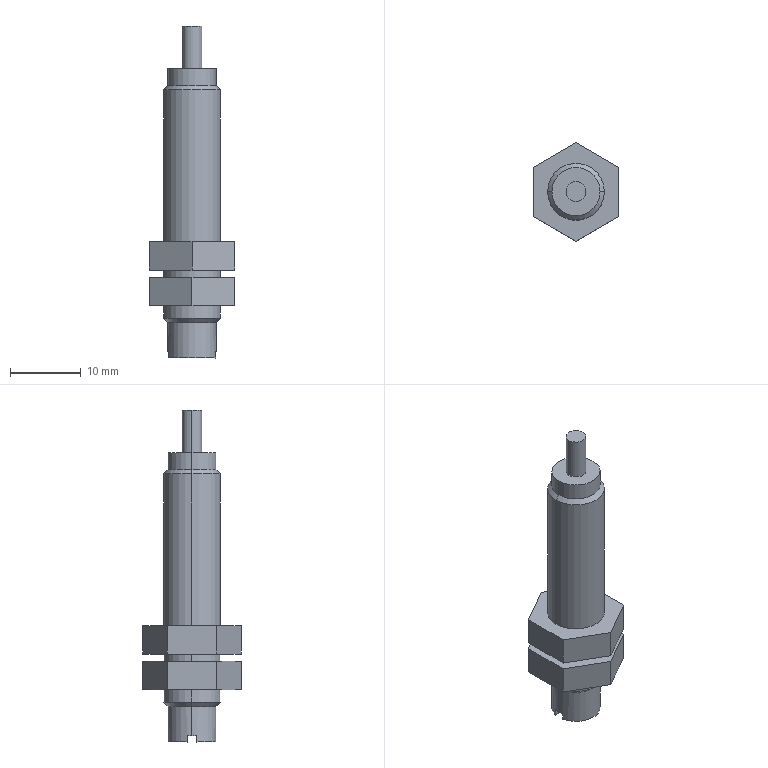Component | SolidWorks | RB0806-2 | 1 solid | 39 faces | box 12 x 13.86 x 46.8 mm | volume 2563 mm3 | plane 23 | cylinder 12 | cone 4 | commonest cylinder face diameters 8 x6 6.8 x4 2.8 x2
STEP:
#1=CARTESIAN_POINT('',(39.223,14.771,-15.48));
#2=VERTEX_POINT('',#1);
#3=CARTESIAN_POINT('',(39.538,14.771,-15.48));
#4=VERTEX_POINT('',#3);
#5=CARTESIAN_POINT('',(39.38,14.771,-15.48));
#6=DIRECTION('',(-0.00002551,-0.,-1.));
#7=DIRECTION('',(-1.,0.,0.00002551));
#8=AXIS2_PLACEMENT_3D('',#5,#6,#7);
#9=CIRCLE('',#8,0.1575);
#10=EDGE_CURVE('',#2,#4,#9,.T.);
#11=ORIENTED_EDGE('',*,*,#10,.F.);
#12=CARTESIAN_POINT('',(39.223,14.771,-14.638));
#13=VERTEX_POINT('',#12);
#14=CARTESIAN_POINT('',(39.223,14.771,-14.638));
#15=DIRECTION('',(0.00002551,0.,1.));
#16=VECTOR('',#15,39.37);
#17=LINE('',#14,#16);
#18=EDGE_CURVE('',#2,#13,#17,.T.);
#19=ORIENTED_EDGE('',*,*,#18,.T.);
#20=CARTESIAN_POINT('',(39.538,14.771,-14.638));
#21=VERTEX_POINT('',#20);
#22=CARTESIAN_POINT('',(39.38,14.771,-14.638));
#23=DIRECTION('',(0.00002551,0.,1.));
#24=DIRECTION('',(0.,1.,0.));
#25=AXIS2_PLACEMENT_3D('',#22,#23,#24);
#26=CIRCLE('',#25,0.1575);
#27=EDGE_CURVE('',#21,#13,#26,.T.);
#28=ORIENTED_EDGE('',*,*,#27,.F.);
#29=CARTESIAN_POINT('',(39.538,14.771,-14.638));
#30=DIRECTION('',(0.00002551,0.,1.));
#31=VECTOR('',#30,39.37);
#32=LINE('',#29,#31);
#33=EDGE_CURVE('',#4,#21,#32,.T.);
#34=ORIENTED_EDGE('',*,*,#33,.F.);
#35=EDGE_LOOP('',(#11,#19,#28,#34));
#36=FACE_OUTER_BOUND('',#35,.T.);
#37=CARTESIAN_POINT('',(39.38,14.771,-14.638));
#38=DIRECTION('',(0.00002551,0.,1.));
#39=DIRECTION('',(1.,0.,-0.00002551));
#40=AXIS2_PLACEMENT_3D('',#37,#38,#39);
#41=CYLINDRICAL_SURFACE('',#40,0.1575);
#42=ADVANCED_FACE('',(#36),#41,.T.);
#43=CARTESIAN_POINT('',(39.514,14.771,-14.614));
#44=VERTEX_POINT('',#43);
#45=CARTESIAN_POINT('',(39.247,14.771,-14.614));
#46=VERTEX_POINT('',#45);
#47=CARTESIAN_POINT('',(39.38,14.771,-14.614));
#48=DIRECTION('',(0.00002551,0.,1.));
#49=DIRECTION('',(0.,1.,0.));
#50=AXIS2_PLACEMENT_3D('',#47,#48,#49);
#51=CIRCLE('',#50,0.1339);
#52=EDGE_CURVE('',#44,#46,#51,.T.);
#53=ORIENTED_EDGE('',*,*,#52,.F.);
#54=CARTESIAN_POINT('',(39.514,14.771,-14.614));
#55=DIRECTION('',(0.7071,-0.,-0.7071));
#56=VECTOR('',#55,39.37);
#57=LINE('',#54,#56);
#58=EDGE_CURVE('',#44,#21,#57,.T.);
#59=ORIENTED_EDGE('',*,*,#58,.T.);
#60=ORIENTED_EDGE('',*,*,#27,.T.);
#61=CARTESIAN_POINT('',(39.247,14.771,-14.614));
#62=DIRECTION('',(-0.7071,-0.,-0.7071));
#63=VECTOR('',#62,39.37);
#64=LINE('',#61,#63);
#65=EDGE_CURVE('',#46,#13,#64,.T.);
#66=ORIENTED_EDGE('',*,*,#65,.F.);
#67=EDGE_LOOP('',(#53,#59,#60,#66));
#68=FACE_OUTER_BOUND('',#67,.T.);
#69=CARTESIAN_POINT('',(39.38,14.771,-14.614));
#70=DIRECTION('',(-0.00002551,-0.,-1.));
#71=DIRECTION('',(-1.,0.,0.00002551));
#72=AXIS2_PLACEMENT_3D('',#69,#70,#71);
#73=CONICAL_SURFACE('',#72,0.1339,0.7854);
#74=ADVANCED_FACE('',(#68),#73,.T.);
#75=ORIENTED_EDGE('',*,*,#52,.T.);
#76=CARTESIAN_POINT('',(39.247,14.771,-14.52));
#77=VERTEX_POINT('',#76);
#78=CARTESIAN_POINT('',(39.247,14.771,-14.52));
#79=DIRECTION('',(0.00002551,0.,1.));
#80=VECTOR('',#79,39.37);
#81=LINE('',#78,#80);
#82=EDGE_CURVE('',#46,#77,#81,.T.);
#83=ORIENTED_EDGE('',*,*,#82,.T.);
#84=CARTESIAN_POINT('',(39.514,14.771,-14.52));
#85=VERTEX_POINT('',#84);
#86=CARTESIAN_POINT('',(39.38,14.771,-14.52));
#87=DIRECTION('',(0.00002551,0.,1.));
#88=DIRECTION('',(1.,0.,-0.00002551));
#89=AXIS2_PLACEMENT_3D('',#86,#87,#88);
#90=CIRCLE('',#89,0.1339);
#91=EDGE_CURVE('',#85,#77,#90,.T.);
#92=ORIENTED_EDGE('',*,*,#91,.F.);
#93=CARTESIAN_POINT('',(39.514,14.771,-14.52));
#94=DIRECTION('',(0.00002551,0.,1.));
#95=VECTOR('',#94,39.37);
#96=LINE('',#93,#95);
#97=EDGE_CURVE('',#44,#85,#96,.T.);
#98=ORIENTED_EDGE('',*,*,#97,.F.);
#99=EDGE_LOOP('',(#75,#83,#92,#98));
#100=FACE_OUTER_BOUND('',#99,.T.);
#101=CARTESIAN_POINT('',(39.38,14.771,-14.52));
#102=DIRECTION('',(0.00002551,0.,1.));
#103=DIRECTION('',(1.,0.,-0.00002551));
#104=AXIS2_PLACEMENT_3D('',#101,#102,#103);
#105=CYLINDRICAL_SURFACE('',#104,0.1339);
#106=ADVANCED_FACE('',(#100),#105,.T.);
#107=CARTESIAN_POINT('',(39.436,14.771,-14.52));
#108=VERTEX_POINT('',#107);
#109=CARTESIAN_POINT('',(39.325,14.771,-14.52));
#110=VERTEX_POINT('',#109);
#111=CARTESIAN_POINT('',(39.38,14.771,-14.52));
#112=DIRECTION('',(0.00002551,0.,1.));
#113=DIRECTION('',(1.,0.,-0.00002551));
#114=AXIS2_PLACEMENT_3D('',#111,#112,#113);
#115=CIRCLE('',#114,0.05512);
#116=EDGE_CURVE('',#108,#110,#115,.T.);
#117=ORIENTED_EDGE('',*,*,#116,.T.);
#118=CARTESIAN_POINT('',(39.325,14.771,-14.283));
#119=VERTEX_POINT('',#118);
#120=CARTESIAN_POINT('',(39.325,14.771,-14.283));
#121=DIRECTION('',(0.00002551,0.,1.));
#122=VECTOR('',#121,39.37);
#123=LINE('',#120,#122);
#124=EDGE_CURVE('',#110,#119,#123,.T.);
#125=ORIENTED_EDGE('',*,*,#124,.T.);
#126=CARTESIAN_POINT('',(39.436,14.771,-14.283));
#127=VERTEX_POINT('',#126);
#128=CARTESIAN_POINT('',(39.38,14.771,-14.283));
#129=DIRECTION('',(-0.00002551,-0.,-1.));
#130=DIRECTION('',(1.,0.,-0.00002551));
#131=AXIS2_PLACEMENT_3D('',#128,#129,#130);
#132=CIRCLE('',#131,0.05512);
#133=EDGE_CURVE('',#119,#127,#132,.T.);
#134=ORIENTED_EDGE('',*,*,#133,.T.);
#135=CARTESIAN_POINT('',(39.436,14.771,-14.283));
#136=DIRECTION('',(0.00002551,0.,1.));
#137=VECTOR('',#136,39.37);
#138=LINE('',#135,#137);
#139=EDGE_CURVE('',#108,#127,#138,.T.);
#140=ORIENTED_EDGE('',*,*,#139,.F.);
#141=EDGE_LOOP('',(#117,#125,#134,#140));
#142=FACE_OUTER_BOUND('',#141,.T.);
#143=CARTESIAN_POINT('',(39.38,14.771,-14.283));
#144=DIRECTION('',(0.00002551,0.,1.));
#145=DIRECTION('',(1.,0.,-0.00002551));
#146=AXIS2_PLACEMENT_3D('',#143,#144,#145);
#147=CYLINDRICAL_SURFACE('',#146,0.05512);
#148=ADVANCED_FACE('',(#142),#147,.T.);
#149=CARTESIAN_POINT('',(39.538,14.771,-15.905));
#150=VERTEX_POINT('',#149);
#151=CARTESIAN_POINT('',(39.223,14.771,-15.905));
#152=VERTEX_POINT('',#151);
#153=CARTESIAN_POINT('',(39.38,14.771,-15.905));
#154=DIRECTION('',(0.00002551,0.,1.));
#155=DIRECTION('',(0.,1.,0.));
#156=AXIS2_PLACEMENT_3D('',#153,#154,#155);
#157=CIRCLE('',#156,0.1575);
#158=EDGE_CURVE('',#150,#152,#157,.T.);
#159=ORIENTED_EDGE('',*,*,#158,.T.);
#160=CARTESIAN_POINT('',(39.223,14.771,-15.835));
#161=VERTEX_POINT('',#160);
#162=CARTESIAN_POINT('',(39.223,14.771,-15.48));
#163=DIRECTION('',(0.00002551,0.,1.));
#164=VECTOR('',#163,39.37);
#165=LINE('',#162,#164);
#166=EDGE_CURVE('',#152,#161,#165,.T.);
#167=ORIENTED_EDGE('',*,*,#166,.T.);
#168=CARTESIAN_POINT('',(39.538,14.771,-15.835));
#169=VERTEX_POINT('',#168);
#170=CARTESIAN_POINT('',(39.38,14.771,-15.835));
#171=DIRECTION('',(-0.00002551,-0.,-1.));
#172=DIRECTION('',(1.,0.,-0.00002551));
#173=AXIS2_PLACEMENT_3D('',#170,#171,#172);
#174=CIRCLE('',#173,0.1575);
#175=EDGE_CURVE('',#161,#169,#174,.T.);
#176=ORIENTED_EDGE('',*,*,#175,.T.);
#177=CARTESIAN_POINT('',(39.538,14.771,-15.48));
#178=DIRECTION('',(0.00002551,0.,1.));
#179=VECTOR('',#178,39.37);
#180=LINE('',#177,#179);
#181=EDGE_CURVE('',#150,#169,#180,.T.);
#182=ORIENTED_EDGE('',*,*,#181,.F.);
#183=EDGE_LOOP('',(#159,#167,#176,#182));
#184=FACE_OUTER_BOUND('',#183,.T.);
#185=CARTESIAN_POINT('',(39.38,14.771,-15.48));
#186=DIRECTION('',(0.00002551,0.,1.));
#187=DIRECTION('',(1.,0.,-0.00002551));
#188=AXIS2_PLACEMENT_3D('',#185,#186,#187);
#189=CYLINDRICAL_SURFACE('',#188,0.1575);
#190=ADVANCED_FACE('',(#184),#189,.T.);
#191=CARTESIAN_POINT('',(39.514,14.771,-15.929));
#192=VERTEX_POINT('',#191);
#193=CARTESIAN_POINT('',(39.247,14.771,-15.929));
#194=VERTEX_POINT('',#193);
#195=CARTESIAN_POINT('',(39.38,14.771,-15.929));
#196=DIRECTION('',(0.00002551,0.,1.));
#197=DIRECTION('',(0.,1.,0.));
#198=AXIS2_PLACEMENT_3D('',#195,#196,#197);
#199=CIRCLE('',#198,0.1339);
#200=EDGE_CURVE('',#192,#194,#199,.T.);
#201=ORIENTED_EDGE('',*,*,#200,.T.);
#202=CARTESIAN_POINT('',(39.247,14.771,-15.929));
#203=DIRECTION('',(-0.7071,0.,0.7071));
#204=VECTOR('',#203,39.37);
#205=LINE('',#202,#204);
#206=EDGE_CURVE('',#194,#152,#205,.T.);
#207=ORIENTED_EDGE('',*,*,#206,.T.);
#208=ORIENTED_EDGE('',*,*,#158,.F.);
#209=CARTESIAN_POINT('',(39.514,14.771,-15.929));
#210=DIRECTION('',(0.7071,0.,0.7071));
#211=VECTOR('',#210,39.37);
#212=LINE('',#209,#211);
#213=EDGE_CURVE('',#192,#150,#212,.T.);
#214=ORIENTED_EDGE('',*,*,#213,.F.);
#215=EDGE_LOOP('',(#201,#207,#208,#214));
#216=FACE_OUTER_BOUND('',#215,.T.);
#217=CARTESIAN_POINT('',(39.38,14.771,-15.929));
#218=DIRECTION('',(0.00002551,0.,1.));
#219=DIRECTION('',(1.,0.,-0.00002551));
#220=AXIS2_PLACEMENT_3D('',#217,#218,#219);
#221=CONICAL_SURFACE('',#220,0.1339,0.7854);
#222=ADVANCED_FACE('',(#216),#221,.T.);
#223=CARTESIAN_POINT('',(39.247,14.771,-16.09));
#224=VERTEX_POINT('',#223);
#225=CARTESIAN_POINT('',(39.249,14.799,-16.09));
#226=VERTEX_POINT('',#225);
#227=CARTESIAN_POINT('',(39.38,14.771,-16.09));
#228=DIRECTION('',(-0.00002551,-0.,-1.));
#229=DIRECTION('',(1.,-0.,-0.00002551));
#230=AXIS2_PLACEMENT_3D('',#227,#228,#229);
#231=CIRCLE('',#230,0.1339);
#232=EDGE_CURVE('',#224,#226,#231,.T.);
#233=ORIENTED_EDGE('',*,*,#232,.F.);
#234=CARTESIAN_POINT('',(39.247,14.771,-15.929));
#235=DIRECTION('',(0.00002551,0.,1.));
#236=VECTOR('',#235,39.37);
#237=LINE('',#234,#236);
#238=EDGE_CURVE('',#224,#194,#237,.T.);
#239=ORIENTED_EDGE('',*,*,#238,.T.);
#240=ORIENTED_EDGE('',*,*,#200,.F.);
#241=CARTESIAN_POINT('',(39.514,14.771,-16.09));
#242=VERTEX_POINT('',#241);
#243=CARTESIAN_POINT('',(39.514,14.771,-15.929));
#244=DIRECTION('',(0.00002551,0.,1.));
#245=VECTOR('',#244,39.37);
#246=LINE('',#243,#245);
#247=EDGE_CURVE('',#242,#192,#246,.T.);
#248=ORIENTED_EDGE('',*,*,#247,.F.);
#249=CARTESIAN_POINT('',(39.511,14.799,-16.09));
#250=VERTEX_POINT('',#249);
#251=CARTESIAN_POINT('',(39.38,14.771,-16.09));
#252=DIRECTION('',(-0.00002551,-0.,-1.));
#253=DIRECTION('',(1.,-0.,-0.00002551));
#254=AXIS2_PLACEMENT_3D('',#251,#252,#253);
#255=CIRCLE('',#254,0.1339);
#256=EDGE_CURVE('',#250,#242,#255,.T.);
#257=ORIENTED_EDGE('',*,*,#256,.F.);
#258=CARTESIAN_POINT('',(39.511,14.799,-16.126));
#259=VERTEX_POINT('',#258);
#260=CARTESIAN_POINT('',(39.511,14.799,-16.108));
#261=DIRECTION('',(0.00002551,0.,1.));
#262=VECTOR('',#261,39.37);
#263=LINE('',#260,#262);
#264=EDGE_CURVE('',#259,#250,#263,.T.);
#265=ORIENTED_EDGE('',*,*,#264,.F.);
#266=CARTESIAN_POINT('',(39.249,14.799,-16.126));
#267=VERTEX_POINT('',#266);
#268=CARTESIAN_POINT('',(39.38,14.771,-16.126));
#269=DIRECTION('',(0.00002551,0.,1.));
#270=DIRECTION('',(1.,0.,-0.00002551));
#271=AXIS2_PLACEMENT_3D('',#268,#269,#270);
#272=CIRCLE('',#271,0.1339);
#273=EDGE_CURVE('',#259,#267,#272,.T.);
#274=ORIENTED_EDGE('',*,*,#273,.T.);
#275=CARTESIAN_POINT('',(39.249,14.799,-16.108));
#276=DIRECTION('',(-0.00002551,-0.,-1.));
#277=VECTOR('',#276,39.37);
#278=LINE('',#275,#277);
#279=EDGE_CURVE('',#226,#267,#278,.T.);
#280=ORIENTED_EDGE('',*,*,#279,.F.);
#281=EDGE_LOOP('',(#233,#239,#240,#248,#257,#265,#274,#280));
#282=FACE_OUTER_BOUND('',#281,.T.);
#283=CARTESIAN_POINT('',(39.38,14.771,-15.929));
#284=DIRECTION('',(0.00002551,0.,1.));
#285=DIRECTION('',(1.,0.,-0.00002551));
#286=AXIS2_PLACEMENT_3D('',#283,#284,#285);
#287=CYLINDRICAL_SURFACE('',#286,0.1339);
#288=ADVANCED_FACE('',(#282),#287,.T.);
#289=CARTESIAN_POINT('',(39.223,14.771,-15.677));
#290=VERTEX_POINT('',#289);
#291=CARTESIAN_POINT('',(39.538,14.771,-15.677));
#292=VERTEX_POINT('',#291);
#293=CARTESIAN_POINT('',(39.38,14.771,-15.677));
#294=DIRECTION('',(-0.00002551,-0.,-1.));
#295=DIRECTION('',(1.,-0.,-0.00002551));
#296=AXIS2_PLACEMENT_3D('',#293,#294,#295);
#297=CIRCLE('',#296,0.1575);
#298=EDGE_CURVE('',#290,#292,#297,.T.);
#299=ORIENTED_EDGE('',*,*,#298,.F.);
#300=CARTESIAN_POINT('',(39.223,14.771,-15.638));
#301=VERTEX_POINT('',#300);
#302=CARTESIAN_POINT('',(39.223,14.771,-15.48));
#303=DIRECTION('',(0.00002551,0.,1.));
#304=VECTOR('',#303,39.37);
#305=LINE('',#302,#304);
#306=EDGE_CURVE('',#290,#301,#305,.T.);
#307=ORIENTED_EDGE('',*,*,#306,.T.);
#308=CARTESIAN_POINT('',(39.538,14.771,-15.638));
#309=VERTEX_POINT('',#308);
#310=CARTESIAN_POINT('',(39.38,14.771,-15.638));
#311=DIRECTION('',(-0.00002551,-0.,-1.));
#312=DIRECTION('',(1.,-0.,-0.00002551));
#313=AXIS2_PLACEMENT_3D('',#310,#311,#312);
#314=CIRCLE('',#313,0.1575);
#315=EDGE_CURVE('',#301,#309,#314,.T.);
#316=ORIENTED_EDGE('',*,*,#315,.T.);
#317=CARTESIAN_POINT('',(39.538,14.771,-15.48));
#318=DIRECTION('',(0.00002551,0.,1.));
#319=VECTOR('',#318,39.37);
#320=LINE('',#317,#319);
#321=EDGE_CURVE('',#292,#309,#320,.T.);
#322=ORIENTED_EDGE('',*,*,#321,.F.);
#323=EDGE_LOOP('',(#299,#307,#316,#322));
#324=FACE_OUTER_BOUND('',#323,.T.);
#325=CARTESIAN_POINT('',(39.38,14.771,-15.48));
#326=DIRECTION('',(0.00002551,0.,1.));
#327=DIRECTION('',(1.,0.,-0.00002551));
#328=AXIS2_PLACEMENT_3D('',#325,#326,#327);
#329=CYLINDRICAL_SURFACE('',#328,0.1575);
#330=ADVANCED_FACE('',(#324),#329,.T.);
#331=CARTESIAN_POINT('',(39.38,15.044,-15.48));
#332=VERTEX_POINT('',#331);
#333=CARTESIAN_POINT('',(39.144,14.908,-15.48));
#334=VERTEX_POINT('',#333);
#335=CARTESIAN_POINT('',(39.144,14.908,-15.48));
#336=DIRECTION('',(-0.866,-0.5,0.00002209));
#337=VECTOR('',#336,39.37);
#338=LINE('',#335,#337);
#339=EDGE_CURVE('',#332,#334,#338,.T.);
#340=ORIENTED_EDGE('',*,*,#339,.F.);
#341=CARTESIAN_POINT('',(39.38,15.044,-15.638));
#342=VERTEX_POINT('',#341);
#343=CARTESIAN_POINT('',(39.38,15.044,-15.323));
#344=DIRECTION('',(-0.00002551,-0.,-1.));
#345=VECTOR('',#344,39.37);
#346=LINE('',#343,#345);
#347=EDGE_CURVE('',#332,#342,#346,.T.);
#348=ORIENTED_EDGE('',*,*,#347,.T.);
#349=CARTESIAN_POINT('',(39.144,14.908,-15.638));
#350=VERTEX_POINT('',#349);
#351=CARTESIAN_POINT('',(39.38,15.044,-15.638));
#352=DIRECTION('',(0.866,0.5,-0.00002209));
#353=VECTOR('',#352,39.37);
#354=LINE('',#351,#353);
#355=EDGE_CURVE('',#350,#342,#354,.T.);
#356=ORIENTED_EDGE('',*,*,#355,.F.);
#357=CARTESIAN_POINT('',(39.144,14.908,-15.323));
#358=DIRECTION('',(0.00002551,0.,1.));
#359=VECTOR('',#358,39.37);
#360=LINE('',#357,#359);
#361=EDGE_CURVE('',#350,#334,#360,.T.);
#362=ORIENTED_EDGE('',*,*,#361,.T.);
#363=EDGE_LOOP('',(#340,#348,#356,#362));
#364=FACE_OUTER_BOUND('',#363,.T.);
#365=CARTESIAN_POINT('',(39.144,14.908,-15.323));
#366=DIRECTION('',(-0.5,0.866,0.00001275));
#367=DIRECTION('',(0.866,0.5,-0.00002209));
#368=AXIS2_PLACEMENT_3D('',#365,#366,#367);
#369=PLANE('',#368);
#370=ADVANCED_FACE('',(#364),#369,.T.);
#371=CARTESIAN_POINT('',(39.617,14.908,-15.48));
#372=VERTEX_POINT('',#371);
#373=CARTESIAN_POINT('',(39.38,15.044,-15.48));
#374=DIRECTION('',(-0.866,0.5,0.00002209));
#375=VECTOR('',#374,39.37);
#376=LINE('',#373,#375);
#377=EDGE_CURVE('',#372,#332,#376,.T.);
#378=ORIENTED_EDGE('',*,*,#377,.F.);
#379=CARTESIAN_POINT('',(39.617,14.908,-15.638));
#380=VERTEX_POINT('',#379);
#381=CARTESIAN_POINT('',(39.617,14.908,-15.323));
#382=DIRECTION('',(-0.00002551,-0.,-1.));
#383=VECTOR('',#382,39.37);
#384=LINE('',#381,#383);
#385=EDGE_CURVE('',#372,#380,#384,.T.);
#386=ORIENTED_EDGE('',*,*,#385,.T.);
#387=CARTESIAN_POINT('',(39.617,14.908,-15.638));
#388=DIRECTION('',(0.866,-0.5,-0.00002209));
#389=VECTOR('',#388,39.37);
#390=LINE('',#387,#389);
#391=EDGE_CURVE('',#342,#380,#390,.T.);
#392=ORIENTED_EDGE('',*,*,#391,.F.);
#393=ORIENTED_EDGE('',*,*,#347,.F.);
#394=EDGE_LOOP('',(#378,#386,#392,#393));
#395=FACE_OUTER_BOUND('',#394,.T.);
#396=CARTESIAN_POINT('',(39.38,15.044,-15.323));
#397=DIRECTION('',(0.5,0.866,-0.00001275));
#398=DIRECTION('',(0.866,-0.5,-0.00002209));
#399=AXIS2_PLACEMENT_3D('',#396,#397,#398);
#400=PLANE('',#399);
#401=ADVANCED_FACE('',(#395),#400,.T.);
#402=CARTESIAN_POINT('',(39.617,14.635,-15.48));
#403=VERTEX_POINT('',#402);
#404=CARTESIAN_POINT('',(39.617,14.908,-15.48));
#405=DIRECTION('',(0.,1.,-0.));
#406=VECTOR('',#405,39.37);
#407=LINE('',#404,#406);
#408=EDGE_CURVE('',#403,#372,#407,.T.);
#409=ORIENTED_EDGE('',*,*,#408,.F.);
#410=CARTESIAN_POINT('',(39.617,14.635,-15.638));
#411=VERTEX_POINT('',#410);
#412=CARTESIAN_POINT('',(39.617,14.635,-15.323));
#413=DIRECTION('',(-0.00002551,-0.,-1.));
#414=VECTOR('',#413,39.37);
#415=LINE('',#412,#414);
#416=EDGE_CURVE('',#403,#411,#415,.T.);
#417=ORIENTED_EDGE('',*,*,#416,.T.);
#418=CARTESIAN_POINT('',(39.617,14.635,-15.638));
#419=DIRECTION('',(-0.,-1.,0.));
#420=VECTOR('',#419,39.37);
#421=LINE('',#418,#420);
#422=EDGE_CURVE('',#380,#411,#421,.T.);
#423=ORIENTED_EDGE('',*,*,#422,.F.);
#424=ORIENTED_EDGE('',*,*,#385,.F.);
#425=EDGE_LOOP('',(#409,#417,#423,#424));
#426=FACE_OUTER_BOUND('',#425,.T.);
#427=CARTESIAN_POINT('',(39.617,14.908,-15.323));
#428=DIRECTION('',(1.,-0.,-0.00002551));
#429=DIRECTION('',(-0.,-1.,0.));
#430=AXIS2_PLACEMENT_3D('',#427,#428,#429);
#431=PLANE('',#430);
#432=ADVANCED_FACE('',(#426),#431,.T.);
#433=CARTESIAN_POINT('',(39.38,14.499,-15.48));
#434=VERTEX_POINT('',#433);
#435=CARTESIAN_POINT('',(39.617,14.635,-15.48));
#436=DIRECTION('',(0.866,0.5,-0.00002209));
#437=VECTOR('',#436,39.37);
#438=LINE('',#435,#437);
#439=EDGE_CURVE('',#434,#403,#438,.T.);
#440=ORIENTED_EDGE('',*,*,#439,.F.);
#441=CARTESIAN_POINT('',(39.38,14.499,-15.638));
#442=VERTEX_POINT('',#441);
#443=CARTESIAN_POINT('',(39.38,14.499,-15.323));
#444=DIRECTION('',(-0.00002551,-0.,-1.));
#445=VECTOR('',#444,39.37);
#446=LINE('',#443,#445);
#447=EDGE_CURVE('',#434,#442,#446,.T.);
#448=ORIENTED_EDGE('',*,*,#447,.T.);
#449=CARTESIAN_POINT('',(39.38,14.499,-15.638));
#450=DIRECTION('',(-0.866,-0.5,0.00002209));
#451=VECTOR('',#450,39.37);
#452=LINE('',#449,#451);
#453=EDGE_CURVE('',#411,#442,#452,.T.);
#454=ORIENTED_EDGE('',*,*,#453,.F.);
#455=ORIENTED_EDGE('',*,*,#416,.F.);
#456=EDGE_LOOP('',(#440,#448,#454,#455));
#457=FACE_OUTER_BOUND('',#456,.T.);
#458=CARTESIAN_POINT('',(39.617,14.635,-15.323));
#459=DIRECTION('',(0.5,-0.866,-0.00001275));
#460=DIRECTION('',(-0.866,-0.5,0.00002209));
#461=AXIS2_PLACEMENT_3D('',#458,#459,#460);
#462=PLANE('',#461);
#463=ADVANCED_FACE('',(#457),#462,.T.);
#464=CARTESIAN_POINT('',(39.144,14.635,-15.48));
#465=VERTEX_POINT('',#464);
#466=CARTESIAN_POINT('',(39.38,14.499,-15.48));
#467=DIRECTION('',(0.866,-0.5,-0.00002209));
#468=VECTOR('',#467,39.37);
#469=LINE('',#466,#468);
#470=EDGE_CURVE('',#465,#434,#469,.T.);
#471=ORIENTED_EDGE('',*,*,#470,.F.);
#472=CARTESIAN_POINT('',(39.144,14.635,-15.638));
#473=VERTEX_POINT('',#472);
#474=CARTESIAN_POINT('',(39.144,14.635,-15.323));
#475=DIRECTION('',(-0.00002551,-0.,-1.));
#476=VECTOR('',#475,39.37);
#477=LINE('',#474,#476);
#478=EDGE_CURVE('',#465,#473,#477,.T.);
#479=ORIENTED_EDGE('',*,*,#478,.T.);
#480=CARTESIAN_POINT('',(39.144,14.635,-15.638));
#481=DIRECTION('',(-0.866,0.5,0.00002209));
#482=VECTOR('',#481,39.37);
#483=LINE('',#480,#482);
#484=EDGE_CURVE('',#442,#473,#483,.T.);
#485=ORIENTED_EDGE('',*,*,#484,.F.);
#486=ORIENTED_EDGE('',*,*,#447,.F.);
#487=EDGE_LOOP('',(#471,#479,#485,#486));
#488=FACE_OUTER_BOUND('',#487,.T.);
#489=CARTESIAN_POINT('',(39.38,14.499,-15.323));
#490=DIRECTION('',(-0.5,-0.866,0.00001275));
#491=DIRECTION('',(-0.866,0.5,0.00002209));
#492=AXIS2_PLACEMENT_3D('',#489,#490,#491);
#493=PLANE('',#492);
#494=ADVANCED_FACE('',(#488),#493,.T.);
#495=CARTESIAN_POINT('',(39.144,14.635,-15.48));
#496=DIRECTION('',(-0.,-1.,0.));
#497=VECTOR('',#496,39.37);
#498=LINE('',#495,#497);
#499=EDGE_CURVE('',#334,#465,#498,.T.);
#500=ORIENTED_EDGE('',*,*,#499,.F.);
#501=ORIENTED_EDGE('',*,*,#361,.F.);
#502=CARTESIAN_POINT('',(39.144,14.908,-15.638));
#503=DIRECTION('',(0.,1.,-0.));
#504=VECTOR('',#503,39.37);
#505=LINE('',#502,#504);
#506=EDGE_CURVE('',#473,#350,#505,.T.);
#507=ORIENTED_EDGE('',*,*,#506,.F.);
#508=ORIENTED_EDGE('',*,*,#478,.F.);
#509=EDGE_LOOP('',(#500,#501,#507,#508));
#510=FACE_OUTER_BOUND('',#509,.T.);
#511=CARTESIAN_POINT('',(39.144,14.635,-15.323));
#512=DIRECTION('',(-1.,0.,0.00002551));
#513=DIRECTION('',(0.,1.,-0.));
#514=AXIS2_PLACEMENT_3D('',#511,#512,#513);
#515=PLANE('',#514);
#516=ADVANCED_FACE('',(#510),#515,.T.);
#517=CARTESIAN_POINT('',(39.38,14.771,-15.638));
#518=DIRECTION('',(-0.00002551,-0.,-1.));
#519=DIRECTION('',(1.,0.,-0.00002551));
#520=AXIS2_PLACEMENT_3D('',#517,#518,#519);
#521=CIRCLE('',#520,0.1575);
#522=EDGE_CURVE('',#309,#301,#521,.T.);
#523=ORIENTED_EDGE('',*,*,#522,.F.);
#524=ORIENTED_EDGE('',*,*,#315,.F.);
#525=EDGE_LOOP('',(#523,#524));
#526=FACE_BOUND('',#525,.T.);
#527=ORIENTED_EDGE('',*,*,#422,.T.);
#528=ORIENTED_EDGE('',*,*,#453,.T.);
#529=ORIENTED_EDGE('',*,*,#484,.T.);
#530=ORIENTED_EDGE('',*,*,#506,.T.);
#531=ORIENTED_EDGE('',*,*,#355,.T.);
#532=ORIENTED_EDGE('',*,*,#391,.T.);
#533=EDGE_LOOP('',(#527,#528,#529,#530,#531,#532));
#534=FACE_OUTER_BOUND('',#533,.T.);
#535=CARTESIAN_POINT('',(39.38,14.771,-15.638));
#536=DIRECTION('',(0.00002551,0.,1.));
#537=DIRECTION('',(1.,-0.,-0.00002551));
#538=AXIS2_PLACEMENT_3D('',#535,#536,#537);
#539=PLANE('',#538);
#540=ADVANCED_FACE('',(#526,#534),#539,.F.);
#541=ORIENTED_EDGE('',*,*,#306,.F.);
#542=CARTESIAN_POINT('',(39.38,14.771,-15.677));
#543=DIRECTION('',(-0.00002551,-0.,-1.));
#544=DIRECTION('',(1.,0.,-0.00002551));
#545=AXIS2_PLACEMENT_3D('',#542,#543,#544);
#546=CIRCLE('',#545,0.1575);
#547=EDGE_CURVE('',#292,#290,#546,.T.);
#548=ORIENTED_EDGE('',*,*,#547,.F.);
#549=ORIENTED_EDGE('',*,*,#321,.T.);
#550=ORIENTED_EDGE('',*,*,#522,.T.);
#551=EDGE_LOOP('',(#541,#548,#549,#550));
#552=FACE_OUTER_BOUND('',#551,.T.);
#553=CARTESIAN_POINT('',(39.38,14.771,-15.48));
#554=DIRECTION('',(0.00002551,0.,1.));
#555=DIRECTION('',(1.,0.,-0.00002551));
#556=AXIS2_PLACEMENT_3D('',#553,#554,#555);
#557=CYLINDRICAL_SURFACE('',#556,0.1575);
#558=ADVANCED_FACE('',(#552),#557,.T.);
#559=CARTESIAN_POINT('',(39.617,14.908,-15.677));
#560=VERTEX_POINT('',#559);
#561=CARTESIAN_POINT('',(39.617,14.635,-15.677));
#562=VERTEX_POINT('',#561);
#563=CARTESIAN_POINT('',(39.617,14.635,-15.677));
#564=DIRECTION('',(-0.,-1.,0.));
#565=VECTOR('',#564,39.37);
#566=LINE('',#563,#565);
#567=EDGE_CURVE('',#560,#562,#566,.T.);
#568=ORIENTED_EDGE('',*,*,#567,.T.);
#569=CARTESIAN_POINT('',(39.617,14.635,-15.835));
#570=VERTEX_POINT('',#569);
#571=CARTESIAN_POINT('',(39.617,14.635,-15.835));
#572=DIRECTION('',(0.00002551,0.,1.));
#573=VECTOR('',#572,39.37);
#574=LINE('',#571,#573);
#575=EDGE_CURVE('',#570,#562,#574,.T.);
#576=ORIENTED_EDGE('',*,*,#575,.F.);
#577=CARTESIAN_POINT('',(39.617,14.908,-15.835));
#578=VERTEX_POINT('',#577);
#579=CARTESIAN_POINT('',(39.617,14.635,-15.835));
#580=DIRECTION('',(-0.,-1.,0.));
#581=VECTOR('',#580,39.37);
#582=LINE('',#579,#581);
#583=EDGE_CURVE('',#578,#570,#582,.T.);
#584=ORIENTED_EDGE('',*,*,#583,.F.);
#585=CARTESIAN_POINT('',(39.617,14.908,-15.835));
#586=DIRECTION('',(0.00002551,0.,1.));
#587=VECTOR('',#586,39.37);
#588=LINE('',#585,#587);
#589=EDGE_CURVE('',#578,#560,#588,.T.);
#590=ORIENTED_EDGE('',*,*,#589,.T.);
#591=EDGE_LOOP('',(#568,#576,#584,#590));
#592=FACE_OUTER_BOUND('',#591,.T.);
#593=CARTESIAN_POINT('',(39.617,14.635,-15.835));
#594=DIRECTION('',(-1.,0.,0.00002551));
#595=DIRECTION('',(-0.,-1.,0.));
#596=AXIS2_PLACEMENT_3D('',#593,#594,#595);
#597=PLANE('',#596);
#598=ADVANCED_FACE('',(#592),#597,.F.);
#599=CARTESIAN_POINT('',(39.38,14.499,-15.677));
#600=VERTEX_POINT('',#599);
#601=CARTESIAN_POINT('',(39.38,14.499,-15.677));
#602=DIRECTION('',(-0.866,-0.5,0.00002209));
#603=VECTOR('',#602,39.37);
#604=LINE('',#601,#603);
#605=EDGE_CURVE('',#562,#600,#604,.T.);
#606=ORIENTED_EDGE('',*,*,#605,.T.);
#607=CARTESIAN_POINT('',(39.38,14.499,-15.835));
#608=VERTEX_POINT('',#607);
#609=CARTESIAN_POINT('',(39.38,14.499,-15.835));
#610=DIRECTION('',(0.00002551,0.,1.));
#611=VECTOR('',#610,39.37);
#612=LINE('',#609,#611);
#613=EDGE_CURVE('',#608,#600,#612,.T.);
#614=ORIENTED_EDGE('',*,*,#613,.F.);
#615=CARTESIAN_POINT('',(39.38,14.499,-15.835));
#616=DIRECTION('',(-0.866,-0.5,0.00002209));
#617=VECTOR('',#616,39.37);
#618=LINE('',#615,#617);
#619=EDGE_CURVE('',#570,#608,#618,.T.);
#620=ORIENTED_EDGE('',*,*,#619,.F.);
#621=ORIENTED_EDGE('',*,*,#575,.T.);
#622=EDGE_LOOP('',(#606,#614,#620,#621));
#623=FACE_OUTER_BOUND('',#622,.T.);
#624=CARTESIAN_POINT('',(39.38,14.499,-15.835));
#625=DIRECTION('',(-0.5,0.866,0.00001275));
#626=DIRECTION('',(-0.866,-0.5,0.00002209));
#627=AXIS2_PLACEMENT_3D('',#624,#625,#626);
#628=PLANE('',#627);
#629=ADVANCED_FACE('',(#623),#628,.F.);
#630=CARTESIAN_POINT('',(39.144,14.635,-15.677));
#631=VERTEX_POINT('',#630);
#632=CARTESIAN_POINT('',(39.144,14.635,-15.677));
#633=DIRECTION('',(-0.866,0.5,0.00002209));
#634=VECTOR('',#633,39.37);
#635=LINE('',#632,#634);
#636=EDGE_CURVE('',#600,#631,#635,.T.);
#637=ORIENTED_EDGE('',*,*,#636,.T.);
#638=CARTESIAN_POINT('',(39.144,14.635,-15.835));
#639=VERTEX_POINT('',#638);
#640=CARTESIAN_POINT('',(39.144,14.635,-15.835));
#641=DIRECTION('',(0.00002551,0.,1.));
#642=VECTOR('',#641,39.37);
#643=LINE('',#640,#642);
#644=EDGE_CURVE('',#639,#631,#643,.T.);
#645=ORIENTED_EDGE('',*,*,#644,.F.);
#646=CARTESIAN_POINT('',(39.144,14.635,-15.835));
#647=DIRECTION('',(-0.866,0.5,0.00002209));
#648=VECTOR('',#647,39.37);
#649=LINE('',#646,#648);
#650=EDGE_CURVE('',#608,#639,#649,.T.);
#651=ORIENTED_EDGE('',*,*,#650,.F.);
#652=ORIENTED_EDGE('',*,*,#613,.T.);
#653=EDGE_LOOP('',(#637,#645,#651,#652));
#654=FACE_OUTER_BOUND('',#653,.T.);
#655=CARTESIAN_POINT('',(39.144,14.635,-15.835));
#656=DIRECTION('',(0.5,0.866,-0.00001275));
#657=DIRECTION('',(-0.866,0.5,0.00002209));
#658=AXIS2_PLACEMENT_3D('',#655,#656,#657);
#659=PLANE('',#658);
#660=ADVANCED_FACE('',(#654),#659,.F.);
#661=CARTESIAN_POINT('',(39.144,14.908,-15.677));
#662=VERTEX_POINT('',#661);
#663=CARTESIAN_POINT('',(39.144,14.908,-15.677));
#664=DIRECTION('',(0.,1.,-0.));
#665=VECTOR('',#664,39.37);
#666=LINE('',#663,#665);
#667=EDGE_CURVE('',#631,#662,#666,.T.);
#668=ORIENTED_EDGE('',*,*,#667,.T.);
#669=CARTESIAN_POINT('',(39.144,14.908,-15.835));
#670=VERTEX_POINT('',#669);
#671=CARTESIAN_POINT('',(39.144,14.908,-15.835));
#672=DIRECTION('',(0.00002551,0.,1.));
#673=VECTOR('',#672,39.37);
#674=LINE('',#671,#673);
#675=EDGE_CURVE('',#670,#662,#674,.T.);
#676=ORIENTED_EDGE('',*,*,#675,.F.);
#677=CARTESIAN_POINT('',(39.144,14.908,-15.835));
#678=DIRECTION('',(0.,1.,-0.));
#679=VECTOR('',#678,39.37);
#680=LINE('',#677,#679);
#681=EDGE_CURVE('',#639,#670,#680,.T.);
#682=ORIENTED_EDGE('',*,*,#681,.F.);
#683=ORIENTED_EDGE('',*,*,#644,.T.);
#684=EDGE_LOOP('',(#668,#676,#682,#683));
#685=FACE_OUTER_BOUND('',#684,.T.);
#686=CARTESIAN_POINT('',(39.144,14.908,-15.835));
#687=DIRECTION('',(1.,-0.,-0.00002551));
#688=DIRECTION('',(0.,1.,-0.));
#689=AXIS2_PLACEMENT_3D('',#686,#687,#688);
#690=PLANE('',#689);
#691=ADVANCED_FACE('',(#685),#690,.F.);
#692=CARTESIAN_POINT('',(39.38,15.044,-15.677));
#693=VERTEX_POINT('',#692);
#694=CARTESIAN_POINT('',(39.38,15.044,-15.677));
#695=DIRECTION('',(0.866,0.5,-0.00002209));
#696=VECTOR('',#695,39.37);
#697=LINE('',#694,#696);
#698=EDGE_CURVE('',#662,#693,#697,.T.);
#699=ORIENTED_EDGE('',*,*,#698,.T.);
#700=CARTESIAN_POINT('',(39.38,15.044,-15.835));
#701=VERTEX_POINT('',#700);
#702=CARTESIAN_POINT('',(39.38,15.044,-15.835));
#703=DIRECTION('',(0.00002551,0.,1.));
#704=VECTOR('',#703,39.37);
#705=LINE('',#702,#704);
#706=EDGE_CURVE('',#701,#693,#705,.T.);
#707=ORIENTED_EDGE('',*,*,#706,.F.);
#708=CARTESIAN_POINT('',(39.38,15.044,-15.835));
#709=DIRECTION('',(0.866,0.5,-0.00002209));
#710=VECTOR('',#709,39.37);
#711=LINE('',#708,#710);
#712=EDGE_CURVE('',#670,#701,#711,.T.);
#713=ORIENTED_EDGE('',*,*,#712,.F.);
#714=ORIENTED_EDGE('',*,*,#675,.T.);
#715=EDGE_LOOP('',(#699,#707,#713,#714));
#716=FACE_OUTER_BOUND('',#715,.T.);
#717=CARTESIAN_POINT('',(39.38,15.044,-15.835));
#718=DIRECTION('',(0.5,-0.866,-0.00001275));
#719=DIRECTION('',(0.866,0.5,-0.00002209));
#720=AXIS2_PLACEMENT_3D('',#717,#718,#719);
#721=PLANE('',#720);
#722=ADVANCED_FACE('',(#716),#721,.F.);
#723=CARTESIAN_POINT('',(39.617,14.908,-15.677));
#724=DIRECTION('',(0.866,-0.5,-0.00002209));
#725=VECTOR('',#724,39.37);
#726=LINE('',#723,#725);
#727=EDGE_CURVE('',#693,#560,#726,.T.);
#728=ORIENTED_EDGE('',*,*,#727,.T.);
#729=ORIENTED_EDGE('',*,*,#589,.F.);
#730=CARTESIAN_POINT('',(39.617,14.908,-15.835));
#731=DIRECTION('',(0.866,-0.5,-0.00002209));
#732=VECTOR('',#731,39.37);
#733=LINE('',#730,#732);
#734=EDGE_CURVE('',#701,#578,#733,.T.);
#735=ORIENTED_EDGE('',*,*,#734,.F.);
#736=ORIENTED_EDGE('',*,*,#706,.T.);
#737=EDGE_LOOP('',(#728,#729,#735,#736));
#738=FACE_OUTER_BOUND('',#737,.T.);
#739=CARTESIAN_POINT('',(39.617,14.908,-15.835));
#740=DIRECTION('',(-0.5,-0.866,0.00001275));
#741=DIRECTION('',(0.866,-0.5,-0.00002209));
#742=AXIS2_PLACEMENT_3D('',#739,#740,#741);
#743=PLANE('',#742);
#744=ADVANCED_FACE('',(#738),#743,.F.);
#745=CARTESIAN_POINT('',(39.38,14.771,-15.835));
#746=DIRECTION('',(-0.00002551,-0.,-1.));
#747=DIRECTION('',(1.,0.,-0.00002551));
#748=AXIS2_PLACEMENT_3D('',#745,#746,#747);
#749=CIRCLE('',#748,0.1575);
#750=EDGE_CURVE('',#169,#161,#749,.T.);
#751=ORIENTED_EDGE('',*,*,#750,.F.);
#752=ORIENTED_EDGE('',*,*,#175,.F.);
#753=EDGE_LOOP('',(#751,#752));
#754=FACE_BOUND('',#753,.T.);
#755=ORIENTED_EDGE('',*,*,#583,.T.);
#756=ORIENTED_EDGE('',*,*,#619,.T.);
#757=ORIENTED_EDGE('',*,*,#650,.T.);
#758=ORIENTED_EDGE('',*,*,#681,.T.);
#759=ORIENTED_EDGE('',*,*,#712,.T.);
#760=ORIENTED_EDGE('',*,*,#734,.T.);
#761=EDGE_LOOP('',(#755,#756,#757,#758,#759,#760));
#762=FACE_OUTER_BOUND('',#761,.T.);
#763=CARTESIAN_POINT('',(39.38,14.771,-15.835));
#764=DIRECTION('',(0.00002551,0.,1.));
#765=DIRECTION('',(1.,-0.,-0.00002551));
#766=AXIS2_PLACEMENT_3D('',#763,#764,#765);
#767=PLANE('',#766);
#768=ADVANCED_FACE('',(#754,#762),#767,.F.);
#769=ORIENTED_EDGE('',*,*,#547,.T.);
#770=ORIENTED_EDGE('',*,*,#298,.T.);
#771=EDGE_LOOP('',(#769,#770));
#772=FACE_BOUND('',#771,.T.);
#773=ORIENTED_EDGE('',*,*,#567,.F.);
#774=ORIENTED_EDGE('',*,*,#727,.F.);
#775=ORIENTED_EDGE('',*,*,#698,.F.);
#776=ORIENTED_EDGE('',*,*,#667,.F.);
#777=ORIENTED_EDGE('',*,*,#636,.F.);
#778=ORIENTED_EDGE('',*,*,#605,.F.);
#779=EDGE_LOOP('',(#773,#774,#775,#776,#777,#778));
#780=FACE_OUTER_BOUND('',#779,.T.);
#781=CARTESIAN_POINT('',(39.38,14.771,-15.677));
#782=DIRECTION('',(0.00002551,0.,1.));
#783=DIRECTION('',(1.,-0.,-0.00002551));
#784=AXIS2_PLACEMENT_3D('',#781,#782,#783);
#785=PLANE('',#784);
#786=ADVANCED_FACE('',(#772,#780),#785,.T.);
#787=CARTESIAN_POINT('',(39.249,14.744,-16.126));
#788=VERTEX_POINT('',#787);
#789=CARTESIAN_POINT('',(39.511,14.744,-16.126));
#790=VERTEX_POINT('',#789);
#791=CARTESIAN_POINT('',(39.38,14.771,-16.126));
#792=DIRECTION('',(0.00002551,0.,1.));
#793=DIRECTION('',(1.,0.,-0.00002551));
#794=AXIS2_PLACEMENT_3D('',#791,#792,#793);
#795=CIRCLE('',#794,0.1339);
#796=EDGE_CURVE('',#788,#790,#795,.T.);
#797=ORIENTED_EDGE('',*,*,#796,.F.);
#798=CARTESIAN_POINT('',(39.511,14.744,-16.126));
#799=DIRECTION('',(1.,-0.,-0.00002551));
#800=VECTOR('',#799,39.37);
#801=LINE('',#798,#800);
#802=EDGE_CURVE('',#788,#790,#801,.T.);
#803=ORIENTED_EDGE('',*,*,#802,.T.);
#804=EDGE_LOOP('',(#797,#803));
#805=FACE_OUTER_BOUND('',#804,.T.);
#806=CARTESIAN_POINT('',(39.513,14.744,-16.126));
#807=DIRECTION('',(-0.00002551,-0.,-1.));
#808=DIRECTION('',(-0.,-1.,0.));
#809=AXIS2_PLACEMENT_3D('',#806,#807,#808);
#810=PLANE('',#809);
#811=ADVANCED_FACE('',(#805),#810,.T.);
#812=CARTESIAN_POINT('',(39.511,14.744,-16.09));
#813=VERTEX_POINT('',#812);
#814=CARTESIAN_POINT('',(39.511,14.744,-16.108));
#815=DIRECTION('',(-0.00002551,-0.,-1.));
#816=VECTOR('',#815,39.37);
#817=LINE('',#814,#816);
#818=EDGE_CURVE('',#813,#790,#817,.T.);
#819=ORIENTED_EDGE('',*,*,#818,.T.);
#820=ORIENTED_EDGE('',*,*,#802,.F.);
#821=CARTESIAN_POINT('',(39.249,14.744,-16.09));
#822=VERTEX_POINT('',#821);
#823=CARTESIAN_POINT('',(39.249,14.744,-16.108));
#824=DIRECTION('',(0.00002551,0.,1.));
#825=VECTOR('',#824,39.37);
#826=LINE('',#823,#825);
#827=EDGE_CURVE('',#788,#822,#826,.T.);
#828=ORIENTED_EDGE('',*,*,#827,.T.);
#829=CARTESIAN_POINT('',(39.511,14.744,-16.09));
#830=DIRECTION('',(1.,-0.,-0.00002551));
#831=VECTOR('',#830,39.37);
#832=LINE('',#829,#831);
#833=EDGE_CURVE('',#822,#813,#832,.T.);
#834=ORIENTED_EDGE('',*,*,#833,.T.);
#835=EDGE_LOOP('',(#819,#820,#828,#834));
#836=FACE_OUTER_BOUND('',#835,.T.);
#837=CARTESIAN_POINT('',(39.511,14.744,-16.09));
#838=DIRECTION('',(0.,1.,-0.));
#839=DIRECTION('',(-0.00002551,-0.,-1.));
#840=AXIS2_PLACEMENT_3D('',#837,#838,#839);
#841=PLANE('',#840);
#842=ADVANCED_FACE('',(#836),#841,.T.);
#843=ORIENTED_EDGE('',*,*,#256,.T.);
#844=CARTESIAN_POINT('',(39.38,14.771,-16.09));
#845=DIRECTION('',(-0.00002551,-0.,-1.));
#846=DIRECTION('',(1.,0.,-0.00002551));
#847=AXIS2_PLACEMENT_3D('',#844,#845,#846);
#848=CIRCLE('',#847,0.1339);
#849=EDGE_CURVE('',#242,#813,#848,.T.);
#850=ORIENTED_EDGE('',*,*,#849,.T.);
#851=ORIENTED_EDGE('',*,*,#833,.F.);
#852=CARTESIAN_POINT('',(39.38,14.771,-16.09));
#853=DIRECTION('',(-0.00002551,-0.,-1.));
#854=DIRECTION('',(1.,-0.,-0.00002551));
#855=AXIS2_PLACEMENT_3D('',#852,#853,#854);
#856=CIRCLE('',#855,0.1339);
#857=EDGE_CURVE('',#822,#224,#856,.T.);
#858=ORIENTED_EDGE('',*,*,#857,.T.);
#859=ORIENTED_EDGE('',*,*,#232,.T.);
#860=CARTESIAN_POINT('',(39.511,14.799,-16.09));
#861=DIRECTION('',(-1.,0.,0.00002551));
#862=VECTOR('',#861,39.37);
#863=LINE('',#860,#862);
#864=EDGE_CURVE('',#250,#226,#863,.T.);
#865=ORIENTED_EDGE('',*,*,#864,.F.);
#866=EDGE_LOOP('',(#843,#850,#851,#858,#859,#865));
#867=FACE_OUTER_BOUND('',#866,.T.);
#868=CARTESIAN_POINT('',(39.516,14.799,-16.09));
#869=DIRECTION('',(-0.00002551,-0.,-1.));
#870=DIRECTION('',(-0.,-1.,0.));
#871=AXIS2_PLACEMENT_3D('',#868,#869,#870);
#872=PLANE('',#871);
#873=ADVANCED_FACE('',(#867),#872,.T.);
#874=CARTESIAN_POINT('',(39.511,14.799,-16.126));
#875=DIRECTION('',(-1.,0.,0.00002551));
#876=VECTOR('',#875,39.37);
#877=LINE('',#874,#876);
#878=EDGE_CURVE('',#259,#267,#877,.T.);
#879=ORIENTED_EDGE('',*,*,#878,.T.);
#880=ORIENTED_EDGE('',*,*,#273,.F.);
#881=EDGE_LOOP('',(#879,#880));
#882=FACE_OUTER_BOUND('',#881,.T.);
#883=CARTESIAN_POINT('',(39.513,14.905,-16.126));
#884=DIRECTION('',(-0.00002551,-0.,-1.));
#885=DIRECTION('',(-0.,-1.,0.));
#886=AXIS2_PLACEMENT_3D('',#883,#884,#885);
#887=PLANE('',#886);
#888=ADVANCED_FACE('',(#882),#887,.T.);
#889=ORIENTED_EDGE('',*,*,#264,.T.);
#890=ORIENTED_EDGE('',*,*,#864,.T.);
#891=ORIENTED_EDGE('',*,*,#279,.T.);
#892=ORIENTED_EDGE('',*,*,#878,.F.);
#893=EDGE_LOOP('',(#889,#890,#891,#892));
#894=FACE_OUTER_BOUND('',#893,.T.);
#895=CARTESIAN_POINT('',(39.511,14.799,-16.126));
#896=DIRECTION('',(-0.,-1.,0.));
#897=DIRECTION('',(0.00002551,0.,1.));
#898=AXIS2_PLACEMENT_3D('',#895,#896,#897);
#899=PLANE('',#898);
#900=ADVANCED_FACE('',(#894),#899,.T.);
#901=ORIENTED_EDGE('',*,*,#238,.F.);
#902=ORIENTED_EDGE('',*,*,#857,.F.);
#903=ORIENTED_EDGE('',*,*,#827,.F.);
#904=ORIENTED_EDGE('',*,*,#796,.T.);
#905=ORIENTED_EDGE('',*,*,#818,.F.);
#906=ORIENTED_EDGE('',*,*,#849,.F.);
#907=ORIENTED_EDGE('',*,*,#247,.T.);
#908=CARTESIAN_POINT('',(39.38,14.771,-15.929));
#909=DIRECTION('',(0.00002551,0.,1.));
#910=DIRECTION('',(0.,1.,0.));
#911=AXIS2_PLACEMENT_3D('',#908,#909,#910);
#912=CIRCLE('',#911,0.1339);
#913=EDGE_CURVE('',#194,#192,#912,.T.);
#914=ORIENTED_EDGE('',*,*,#913,.F.);
#915=EDGE_LOOP('',(#901,#902,#903,#904,#905,#906,#907,#914));
#916=FACE_OUTER_BOUND('',#915,.T.);
#917=CARTESIAN_POINT('',(39.38,14.771,-15.929));
#918=DIRECTION('',(0.00002551,0.,1.));
#919=DIRECTION('',(1.,0.,-0.00002551));
#920=AXIS2_PLACEMENT_3D('',#917,#918,#919);
#921=CYLINDRICAL_SURFACE('',#920,0.1339);
#922=ADVANCED_FACE('',(#916),#921,.T.);
#923=ORIENTED_EDGE('',*,*,#206,.F.);
#924=ORIENTED_EDGE('',*,*,#913,.T.);
#925=ORIENTED_EDGE('',*,*,#213,.T.);
#926=CARTESIAN_POINT('',(39.38,14.771,-15.905));
#927=DIRECTION('',(0.00002551,0.,1.));
#928=DIRECTION('',(0.,1.,0.));
#929=AXIS2_PLACEMENT_3D('',#926,#927,#928);
#930=CIRCLE('',#929,0.1575);
#931=EDGE_CURVE('',#152,#150,#930,.T.);
#932=ORIENTED_EDGE('',*,*,#931,.F.);
#933=EDGE_LOOP('',(#923,#924,#925,#932));
#934=FACE_OUTER_BOUND('',#933,.T.);
#935=CARTESIAN_POINT('',(39.38,14.771,-15.929));
#936=DIRECTION('',(0.00002551,0.,1.));
#937=DIRECTION('',(1.,0.,-0.00002551));
#938=AXIS2_PLACEMENT_3D('',#935,#936,#937);
#939=CONICAL_SURFACE('',#938,0.1339,0.7854);
#940=ADVANCED_FACE('',(#934),#939,.T.);
#941=ORIENTED_EDGE('',*,*,#166,.F.);
#942=ORIENTED_EDGE('',*,*,#931,.T.);
#943=ORIENTED_EDGE('',*,*,#181,.T.);
#944=ORIENTED_EDGE('',*,*,#750,.T.);
#945=EDGE_LOOP('',(#941,#942,#943,#944));
#946=FACE_OUTER_BOUND('',#945,.T.);
#947=CARTESIAN_POINT('',(39.38,14.771,-15.48));
#948=DIRECTION('',(0.00002551,0.,1.));
#949=DIRECTION('',(1.,0.,-0.00002551));
#950=AXIS2_PLACEMENT_3D('',#947,#948,#949);
#951=CYLINDRICAL_SURFACE('',#950,0.1575);
#952=ADVANCED_FACE('',(#946),#951,.T.);
#953=ORIENTED_EDGE('',*,*,#499,.T.);
#954=ORIENTED_EDGE('',*,*,#470,.T.);
#955=ORIENTED_EDGE('',*,*,#439,.T.);
#956=ORIENTED_EDGE('',*,*,#408,.T.);
#957=ORIENTED_EDGE('',*,*,#377,.T.);
#958=ORIENTED_EDGE('',*,*,#339,.T.);
#959=EDGE_LOOP('',(#953,#954,#955,#956,#957,#958));
#960=FACE_OUTER_BOUND('',#959,.T.);
#961=CARTESIAN_POINT('',(39.38,14.771,-15.48));
#962=DIRECTION('',(-0.00002551,-0.,-1.));
#963=DIRECTION('',(-1.,0.,0.00002551));
#964=AXIS2_PLACEMENT_3D('',#961,#962,#963);
#965=CIRCLE('',#964,0.1575);
#966=EDGE_CURVE('',#4,#2,#965,.T.);
#967=ORIENTED_EDGE('',*,*,#966,.T.);
#968=ORIENTED_EDGE('',*,*,#10,.T.);
#969=EDGE_LOOP('',(#967,#968));
#970=FACE_BOUND('',#969,.T.);
#971=CARTESIAN_POINT('',(39.38,14.771,-15.48));
#972=DIRECTION('',(-0.00002551,-0.,-1.));
#973=DIRECTION('',(-1.,0.,0.00002551));
#974=AXIS2_PLACEMENT_3D('',#971,#972,#973);
#975=PLANE('',#974);
#976=ADVANCED_FACE('',(#960,#970),#975,.F.);
#977=CARTESIAN_POINT('',(39.38,14.771,-14.283));
#978=DIRECTION('',(-0.00002551,-0.,-1.));
#979=DIRECTION('',(1.,0.,-0.00002551));
#980=AXIS2_PLACEMENT_3D('',#977,#978,#979);
#981=CIRCLE('',#980,0.05512);
#982=EDGE_CURVE('',#127,#119,#981,.T.);
#983=ORIENTED_EDGE('',*,*,#982,.F.);
#984=ORIENTED_EDGE('',*,*,#133,.F.);
#985=EDGE_LOOP('',(#983,#984));
#986=FACE_OUTER_BOUND('',#985,.T.);
#987=CARTESIAN_POINT('',(39.436,14.716,-14.283));
#988=DIRECTION('',(0.00002551,0.,1.));
#989=DIRECTION('',(0.,1.,-0.));
#990=AXIS2_PLACEMENT_3D('',#987,#988,#989);
#991=PLANE('',#990);
#992=ADVANCED_FACE('',(#986),#991,.T.);
#993=ORIENTED_EDGE('',*,*,#124,.F.);
#994=CARTESIAN_POINT('',(39.38,14.771,-14.52));
#995=DIRECTION('',(0.00002551,0.,1.));
#996=DIRECTION('',(1.,0.,-0.00002551));
#997=AXIS2_PLACEMENT_3D('',#994,#995,#996);
#998=CIRCLE('',#997,0.05512);
#999=EDGE_CURVE('',#110,#108,#998,.T.);
#1000=ORIENTED_EDGE('',*,*,#999,.T.);
#1001=ORIENTED_EDGE('',*,*,#139,.T.);
#1002=ORIENTED_EDGE('',*,*,#982,.T.);
#1003=EDGE_LOOP('',(#993,#1000,#1001,#1002));
#1004=FACE_OUTER_BOUND('',#1003,.T.);
#1005=CARTESIAN_POINT('',(39.38,14.771,-14.283));
#1006=DIRECTION('',(0.00002551,0.,1.));
#1007=DIRECTION('',(1.,0.,-0.00002551));
#1008=AXIS2_PLACEMENT_3D('',#1005,#1006,#1007);
#1009=CYLINDRICAL_SURFACE('',#1008,0.05512);
#1010=ADVANCED_FACE('',(#1004),#1009,.T.);
#1011=ORIENTED_EDGE('',*,*,#116,.F.);
#1012=ORIENTED_EDGE('',*,*,#999,.F.);
#1013=EDGE_LOOP('',(#1011,#1012));
#1014=FACE_BOUND('',#1013,.T.);
#1015=ORIENTED_EDGE('',*,*,#91,.T.);
#1016=CARTESIAN_POINT('',(39.38,14.771,-14.52));
#1017=DIRECTION('',(0.00002551,0.,1.));
#1018=DIRECTION('',(1.,0.,-0.00002551));
#1019=AXIS2_PLACEMENT_3D('',#1016,#1017,#1018);
#1020=CIRCLE('',#1019,0.1339);
#1021=EDGE_CURVE('',#77,#85,#1020,.T.);
#1022=ORIENTED_EDGE('',*,*,#1021,.T.);
#1023=EDGE_LOOP('',(#1015,#1022));
#1024=FACE_OUTER_BOUND('',#1023,.T.);
#1025=CARTESIAN_POINT('',(39.516,14.638,-14.52));
#1026=DIRECTION('',(0.00002551,0.,1.));
#1027=DIRECTION('',(0.,1.,-0.));
#1028=AXIS2_PLACEMENT_3D('',#1025,#1026,#1027);
#1029=PLANE('',#1028);
#1030=ADVANCED_FACE('',(#1014,#1024),#1029,.T.);
#1031=ORIENTED_EDGE('',*,*,#82,.F.);
#1032=CARTESIAN_POINT('',(39.38,14.771,-14.614));
#1033=DIRECTION('',(0.00002551,0.,1.));
#1034=DIRECTION('',(0.,1.,0.));
#1035=AXIS2_PLACEMENT_3D('',#1032,#1033,#1034);
#1036=CIRCLE('',#1035,0.1339);
#1037=EDGE_CURVE('',#46,#44,#1036,.T.);
#1038=ORIENTED_EDGE('',*,*,#1037,.T.);
#1039=ORIENTED_EDGE('',*,*,#97,.T.);
#1040=ORIENTED_EDGE('',*,*,#1021,.F.);
#1041=EDGE_LOOP('',(#1031,#1038,#1039,#1040));
#1042=FACE_OUTER_BOUND('',#1041,.T.);
#1043=CARTESIAN_POINT('',(39.38,14.771,-14.52));
#1044=DIRECTION('',(0.00002551,0.,1.));
#1045=DIRECTION('',(1.,0.,-0.00002551));
#1046=AXIS2_PLACEMENT_3D('',#1043,#1044,#1045);
#1047=CYLINDRICAL_SURFACE('',#1046,0.1339);
#1048=ADVANCED_FACE('',(#1042),#1047,.T.);
#1049=ORIENTED_EDGE('',*,*,#58,.F.);
#1050=ORIENTED_EDGE('',*,*,#1037,.F.);
#1051=ORIENTED_EDGE('',*,*,#65,.T.);
#1052=CARTESIAN_POINT('',(39.38,14.771,-14.638));
#1053=DIRECTION('',(0.00002551,0.,1.));
#1054=DIRECTION('',(0.,1.,0.));
#1055=AXIS2_PLACEMENT_3D('',#1052,#1053,#1054);
#1056=CIRCLE('',#1055,0.1575);
#1057=EDGE_CURVE('',#13,#21,#1056,.T.);
#1058=ORIENTED_EDGE('',*,*,#1057,.T.);
#1059=EDGE_LOOP('',(#1049,#1050,#1051,#1058));
#1060=FACE_OUTER_BOUND('',#1059,.T.);
#1061=CARTESIAN_POINT('',(39.38,14.771,-14.614));
#1062=DIRECTION('',(-0.00002551,-0.,-1.));
#1063=DIRECTION('',(-1.,0.,0.00002551));
#1064=AXIS2_PLACEMENT_3D('',#1061,#1062,#1063);
#1065=CONICAL_SURFACE('',#1064,0.1339,0.7854);
#1066=ADVANCED_FACE('',(#1060),#1065,.T.);
#1067=ORIENTED_EDGE('',*,*,#18,.F.);
#1068=ORIENTED_EDGE('',*,*,#966,.F.);
#1069=ORIENTED_EDGE('',*,*,#33,.T.);
#1070=ORIENTED_EDGE('',*,*,#1057,.F.);
#1071=EDGE_LOOP('',(#1067,#1068,#1069,#1070));
#1072=FACE_OUTER_BOUND('',#1071,.T.);
#1073=CARTESIAN_POINT('',(39.38,14.771,-14.638));
#1074=DIRECTION('',(0.00002551,0.,1.));
#1075=DIRECTION('',(1.,0.,-0.00002551));
#1076=AXIS2_PLACEMENT_3D('',#1073,#1074,#1075);
#1077=CYLINDRICAL_SURFACE('',#1076,0.1575);
#1078=ADVANCED_FACE('',(#1072),#1077,.T.);
#1079=CLOSED_SHELL('',(#42,#74,#106,#148,#190,#222,#288,#330,#370,#401,#432,#463,#494,#516,#540,#558,#598,#629,#660,#691,#722,#744,#768,#786,#811,#842,#873,#888,#900,#922,#940,#952,#976,#992,#1010,#1030,#1048,#1066,#1078));
#1080=MANIFOLD_SOLID_BREP('',#1079);
#1081=CARTESIAN_POINT('',(0.,0.,0.));
#1082=DIRECTION('',(0.,0.,1.));
#1083=DIRECTION('',(1.,0.,0.));
#1084=AXIS2_PLACEMENT_3D('',#1081,#1082,#1083);
#1085=(LENGTH_UNIT()NAMED_UNIT(*)SI_UNIT($,.METRE.));
#1086=LENGTH_MEASURE_WITH_UNIT(LENGTH_MEASURE(0.0254),#1085);
#1087=DIMENSIONAL_EXPONENTS(1.,0.,0.,0.,0.,0.,0.);
#1088=(CONVERSION_BASED_UNIT('',#1086)LENGTH_UNIT()NAMED_UNIT(#1087));
#1089=UNCERTAINTY_MEASURE_WITH_UNIT(LENGTH_MEASURE(0.00001),#1088,'','');
#1090=(NAMED_UNIT(*)PLANE_ANGLE_UNIT()SI_UNIT($,.RADIAN.));
#1091=(NAMED_UNIT(*)SI_UNIT($,.STERADIAN.)SOLID_ANGLE_UNIT());
#1092=(GEOMETRIC_REPRESENTATION_CONTEXT(3)GLOBAL_UNCERTAINTY_ASSIGNED_CONTEXT((#1089))GLOBAL_UNIT_ASSIGNED_CONTEXT((#1088,#1090,#1091))REPRESENTATION_CONTEXT('',''));
#1093=ADVANCED_BREP_SHAPE_REPRESENTATION('',(#1080,#1084),#1092);
#1094=COLOUR_RGB('',0.7922,0.8196,0.9333);
#1095=FILL_AREA_STYLE_COLOUR('',#1094);
#1096=FILL_AREA_STYLE('',(#1095));
#1097=SURFACE_STYLE_FILL_AREA(#1096);
#1098=SURFACE_SIDE_STYLE('',(#1097));
#1099=SURFACE_STYLE_USAGE(.BOTH.,#1098);
#1100=PRESENTATION_STYLE_ASSIGNMENT((#1099));
#1101=STYLED_ITEM('',(#1100),#1080);
#1102=PRESENTATION_LAYER_ASSIGNMENT('','',(#1101));
#1103=(LENGTH_UNIT()NAMED_UNIT(*)SI_UNIT($,.METRE.));
#1104=LENGTH_MEASURE_WITH_UNIT(LENGTH_MEASURE(0.0254),#1103);
#1105=DIMENSIONAL_EXPONENTS(1.,0.,0.,0.,0.,0.,0.);
#1106=(CONVERSION_BASED_UNIT('',#1104)LENGTH_UNIT()NAMED_UNIT(#1105));
#1107=UNCERTAINTY_MEASURE_WITH_UNIT(LENGTH_MEASURE(0.00001),#1106,'','');
#1108=(NAMED_UNIT(*)PLANE_ANGLE_UNIT()SI_UNIT($,.RADIAN.));
#1109=(NAMED_UNIT(*)SI_UNIT($,.STERADIAN.)SOLID_ANGLE_UNIT());
#1110=(GEOMETRIC_REPRESENTATION_CONTEXT(3)GLOBAL_UNCERTAINTY_ASSIGNED_CONTEXT((#1107))GLOBAL_UNIT_ASSIGNED_CONTEXT((#1106,#1108,#1109))REPRESENTATION_CONTEXT('',''));
#1111=MECHANICAL_DESIGN_GEOMETRIC_PRESENTATION_REPRESENTATION('',(#1101),#1110);